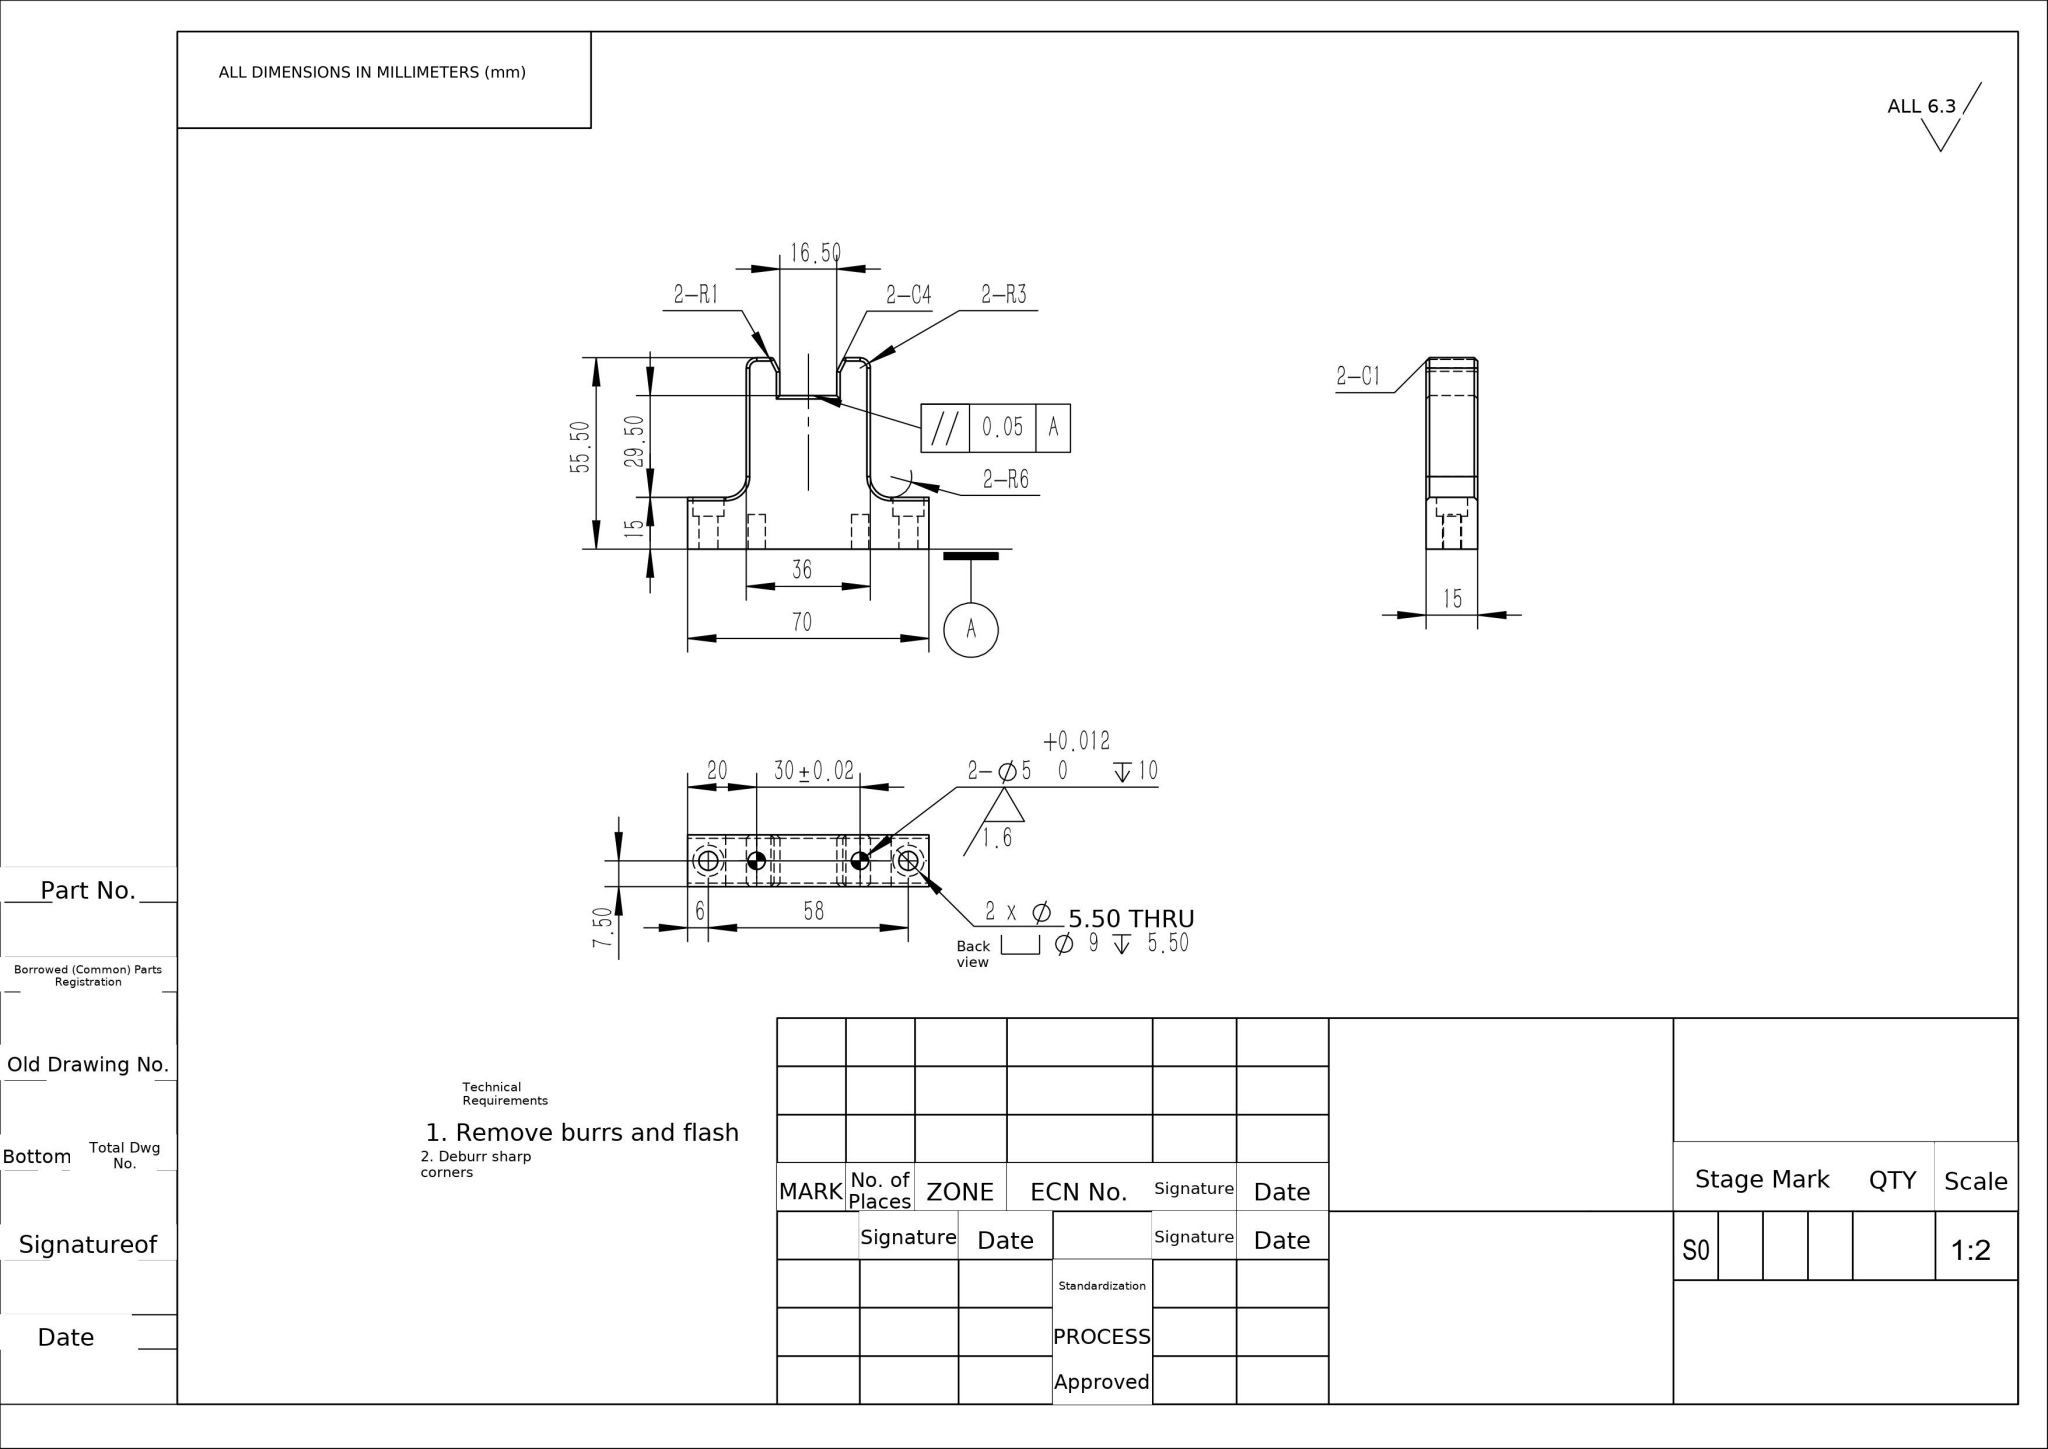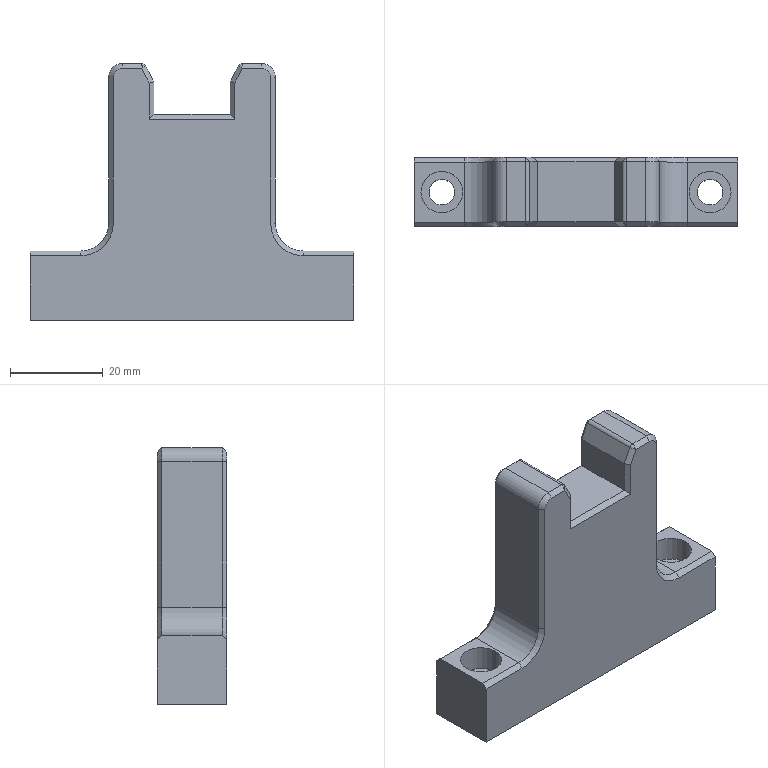Part | NX | mm | 1 solid | 72 faces | box 70 x 15 x 55.5 mm | volume 33243 mm3 | plane 42 | cylinder 18 | cone 12 | commonest cylinder face diameters 5.5 x4 9 x4 5 x4 12 x2 6 x2 2 x2